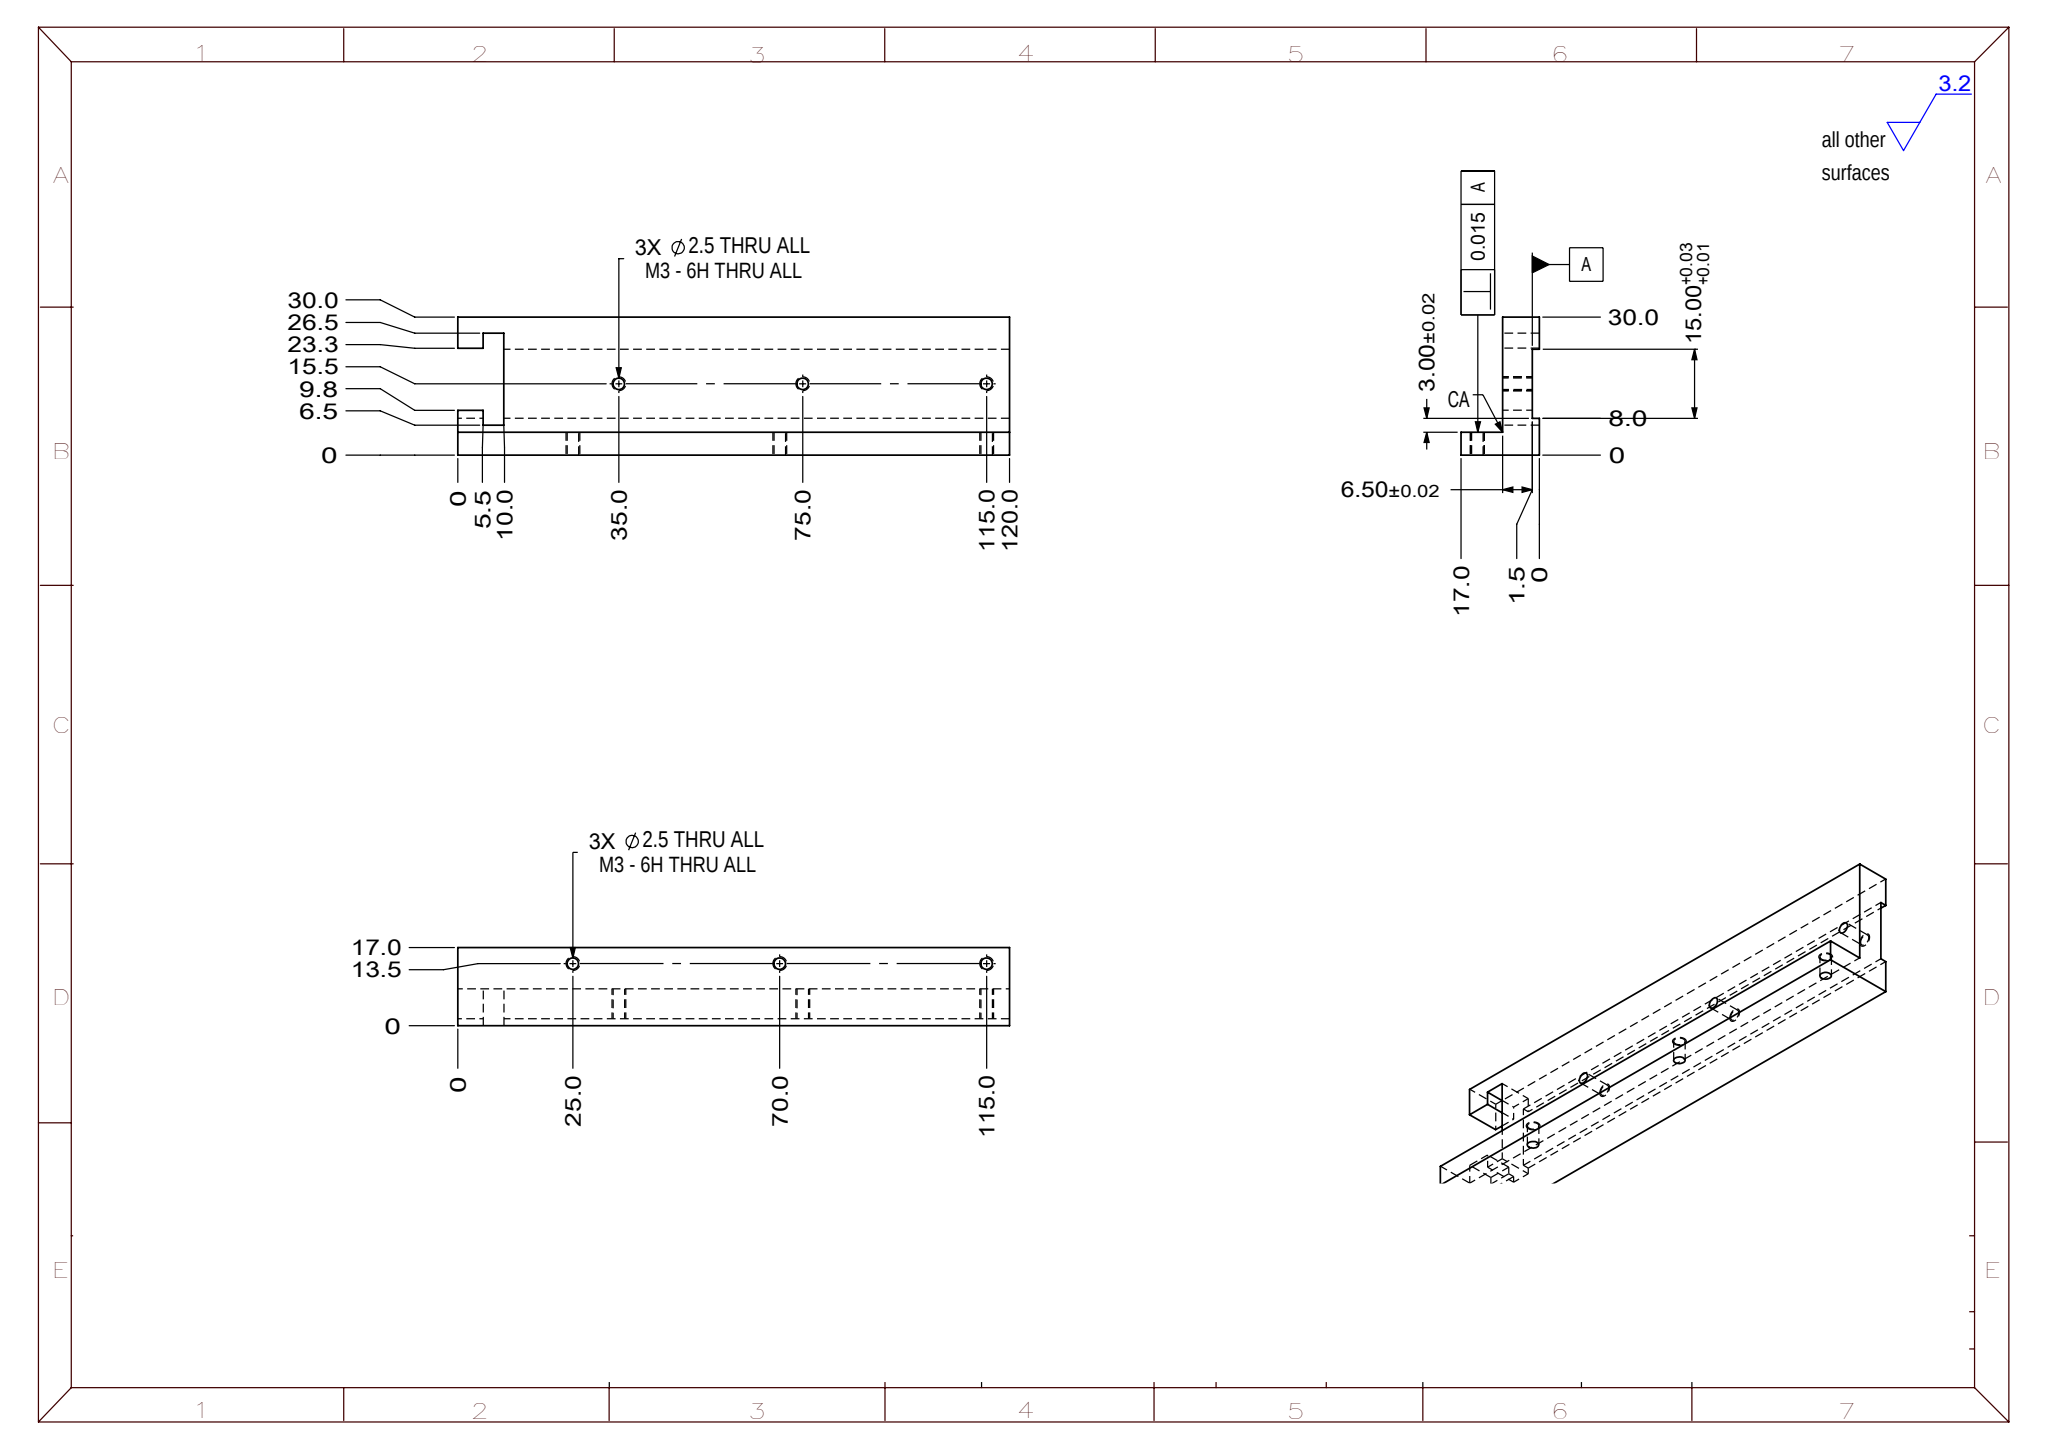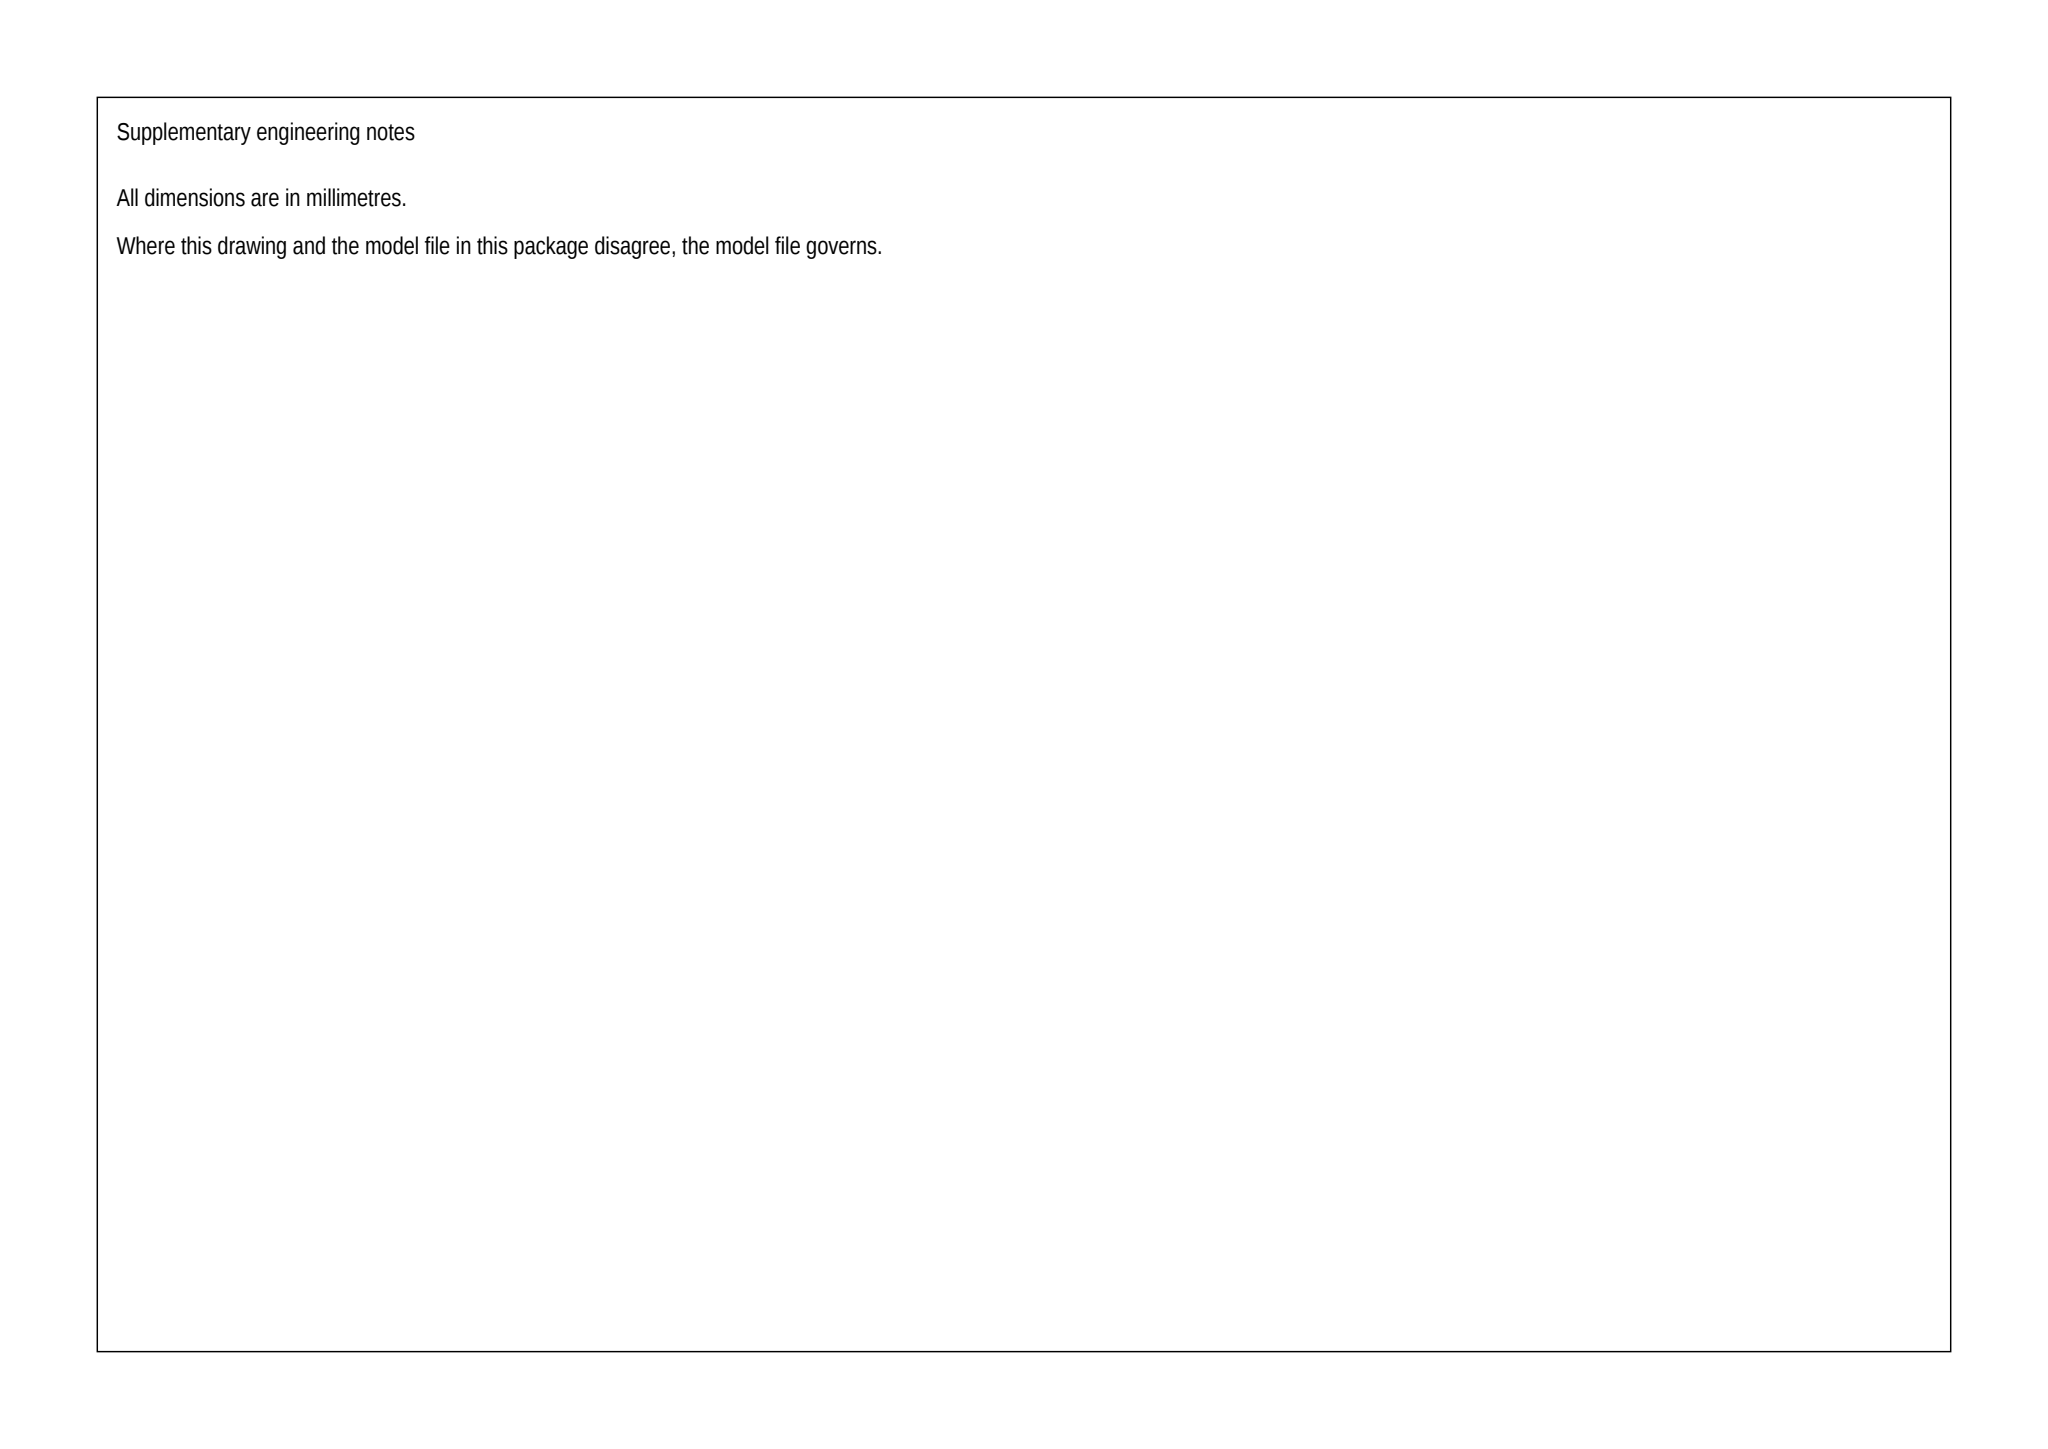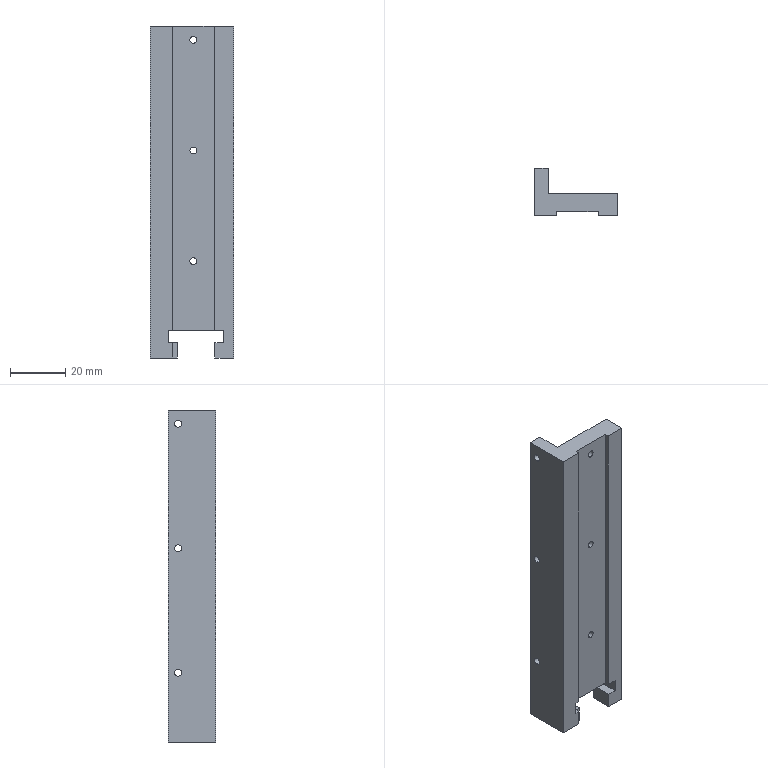Part | SolidWorks | mm | 1 solid | 34 faces | box 30 x 17 x 120 mm | volume 30227 mm3 | plane 22 | cylinder 12 | commonest cylinder face diameters 2.5 x12
Drawing notes:
STOCK ENVELOPE 120.0 LG X 30.0 X 17.0 | from the solid: bbox_xyz [30.0, 17.0, 120.0]
CHANNEL: SIDE WALLS 5.0 & 3.5 THK (X0-5.0, X26.5-30.0); WEB 6.5 THK (Y1.5-8.0) | from the solid: x planes 0/5.0/26.5/30.0; y planes 0/1.5/8.0/17.0; hole lengths 5.0 and 6.5
Z0 END STEPS 5.5 & 10.0 WIDE; 3.5 DP FR X30, 6.5 DP FR X0 | from the solid: z planes 0/5.5/10.0; x planes 0/6.5/26.5/30.0
3X M3-6H THRU, Ø2.5 PILOT THRU 6.5 WEB, CL X15.5, Z 35/75/115 FR Z0 | from the solid: cylinders Ø2.5 axis y at x=15.5, z=35/75/115, length 6.5
3X M3-6H THRU, Ø2.5 PILOT THRU 5.0 WALL, CL Y13.5, Z 25/70/115 FR Z0 | from the solid: cylinders Ø2.5 axis x at y=13.5, z=25/70/115, length 5.0
3X M3-6H THRU, Ø2.5 PILOT THRU 6.5 WEB; HOLE CL X15.5 FROM X0, Z 35.0 / 75.0 / 115.0 FROM Z0 | from the solid: cylinders dia 2.5, axis y, pos [15.5, -, 35.0/75.0/115.0], length 6.5
3X Ø2.5 THRU 6.5 WEB, TAP M3-6H THRU; HOLE CL 15.5 FROM X0, AT Z 35.0/75.0/115.0 FROM Z0 | from the solid: cylinders [2.5,"y",[15.5,null,35.0],6.5], [2.5,"y",[15.5,null,75.0],6.5], [2.5,"y",[15.5,null,115.0],6.5]
3X M3-6H THRU, Ø2.5 PILOT THRU 6.5 WEB, CL 15.5 FROM X0, AT Z 35.0 / 75.0 / 115.0 FROM Z0 | from the solid: cylinders [2.5,"y",[15.5,null,35.0],6.5], [2.5,"y",[15.5,null,75.0],6.5], [2.5,"y",[15.5,null,115.0],6.5]
build123d program:
from build123d import *

# Parameters (mm, degrees)
BOSS_EXTRUDE1_DEPTH = 60
CUT_EXTRUDE1_DEPTH  = 63.498
M3_TAPPED_HOLE1_D   = 2.5
M3_TAPPED_HOLE2_D   = 2.5


with BuildPart() as part:
    # Sketch1 → Boss-Extrude1 (new, symmetric)
    with BuildSketch(Plane.XY):
        Polygon((-10, 8.5), (-10, -0.5), (15, -0.5), (15, -8.5), (8, -8.5), (8, -7), (-7, -7), (-7, -8.5), (-15, -8.5), (-15, 8.5), align=None)
    extrude(amount=BOSS_EXTRUDE1_DEPTH, both=True)

    # Sketch2 → Cut-Extrude1 (cut, through all)
    with BuildSketch(Plane(origin=(0, -0.5, 0), x_dir=(1, 0, 0), z_dir=(0, 1, 0))):
        Polygon((11.5, 54.5), (8.25, 54.5), (8.25, 60), (-5.25, 60), (-5.25, 54.5), (-8.5, 54.5), (-8.5, 50), (11.5, 50), align=None)
    extrude(amount=-CUT_EXTRUDE1_DEPTH, mode=Mode.SUBTRACT)

    # M3 Tapped Hole1 (through all)
    with Locations(Plane(origin=(0, -7, 0), x_dir=(-1, 0, 0), z_dir=(0, -1, 0))):
        with Locations((-0.5, -55), (-0.5, -15), (-0.5, 25)):
            Hole(M3_TAPPED_HOLE1_D / 2)

    # M3 Tapped Hole2 (through all)
    with Locations(Plane(origin=(-10, 0, 0), x_dir=(0, 0, -1), z_dir=(1, 0, 0))):
        with Locations((-55, 5), (-10, 5), (35, 5)):
            Hole(M3_TAPPED_HOLE2_D / 2)


solid = part.part